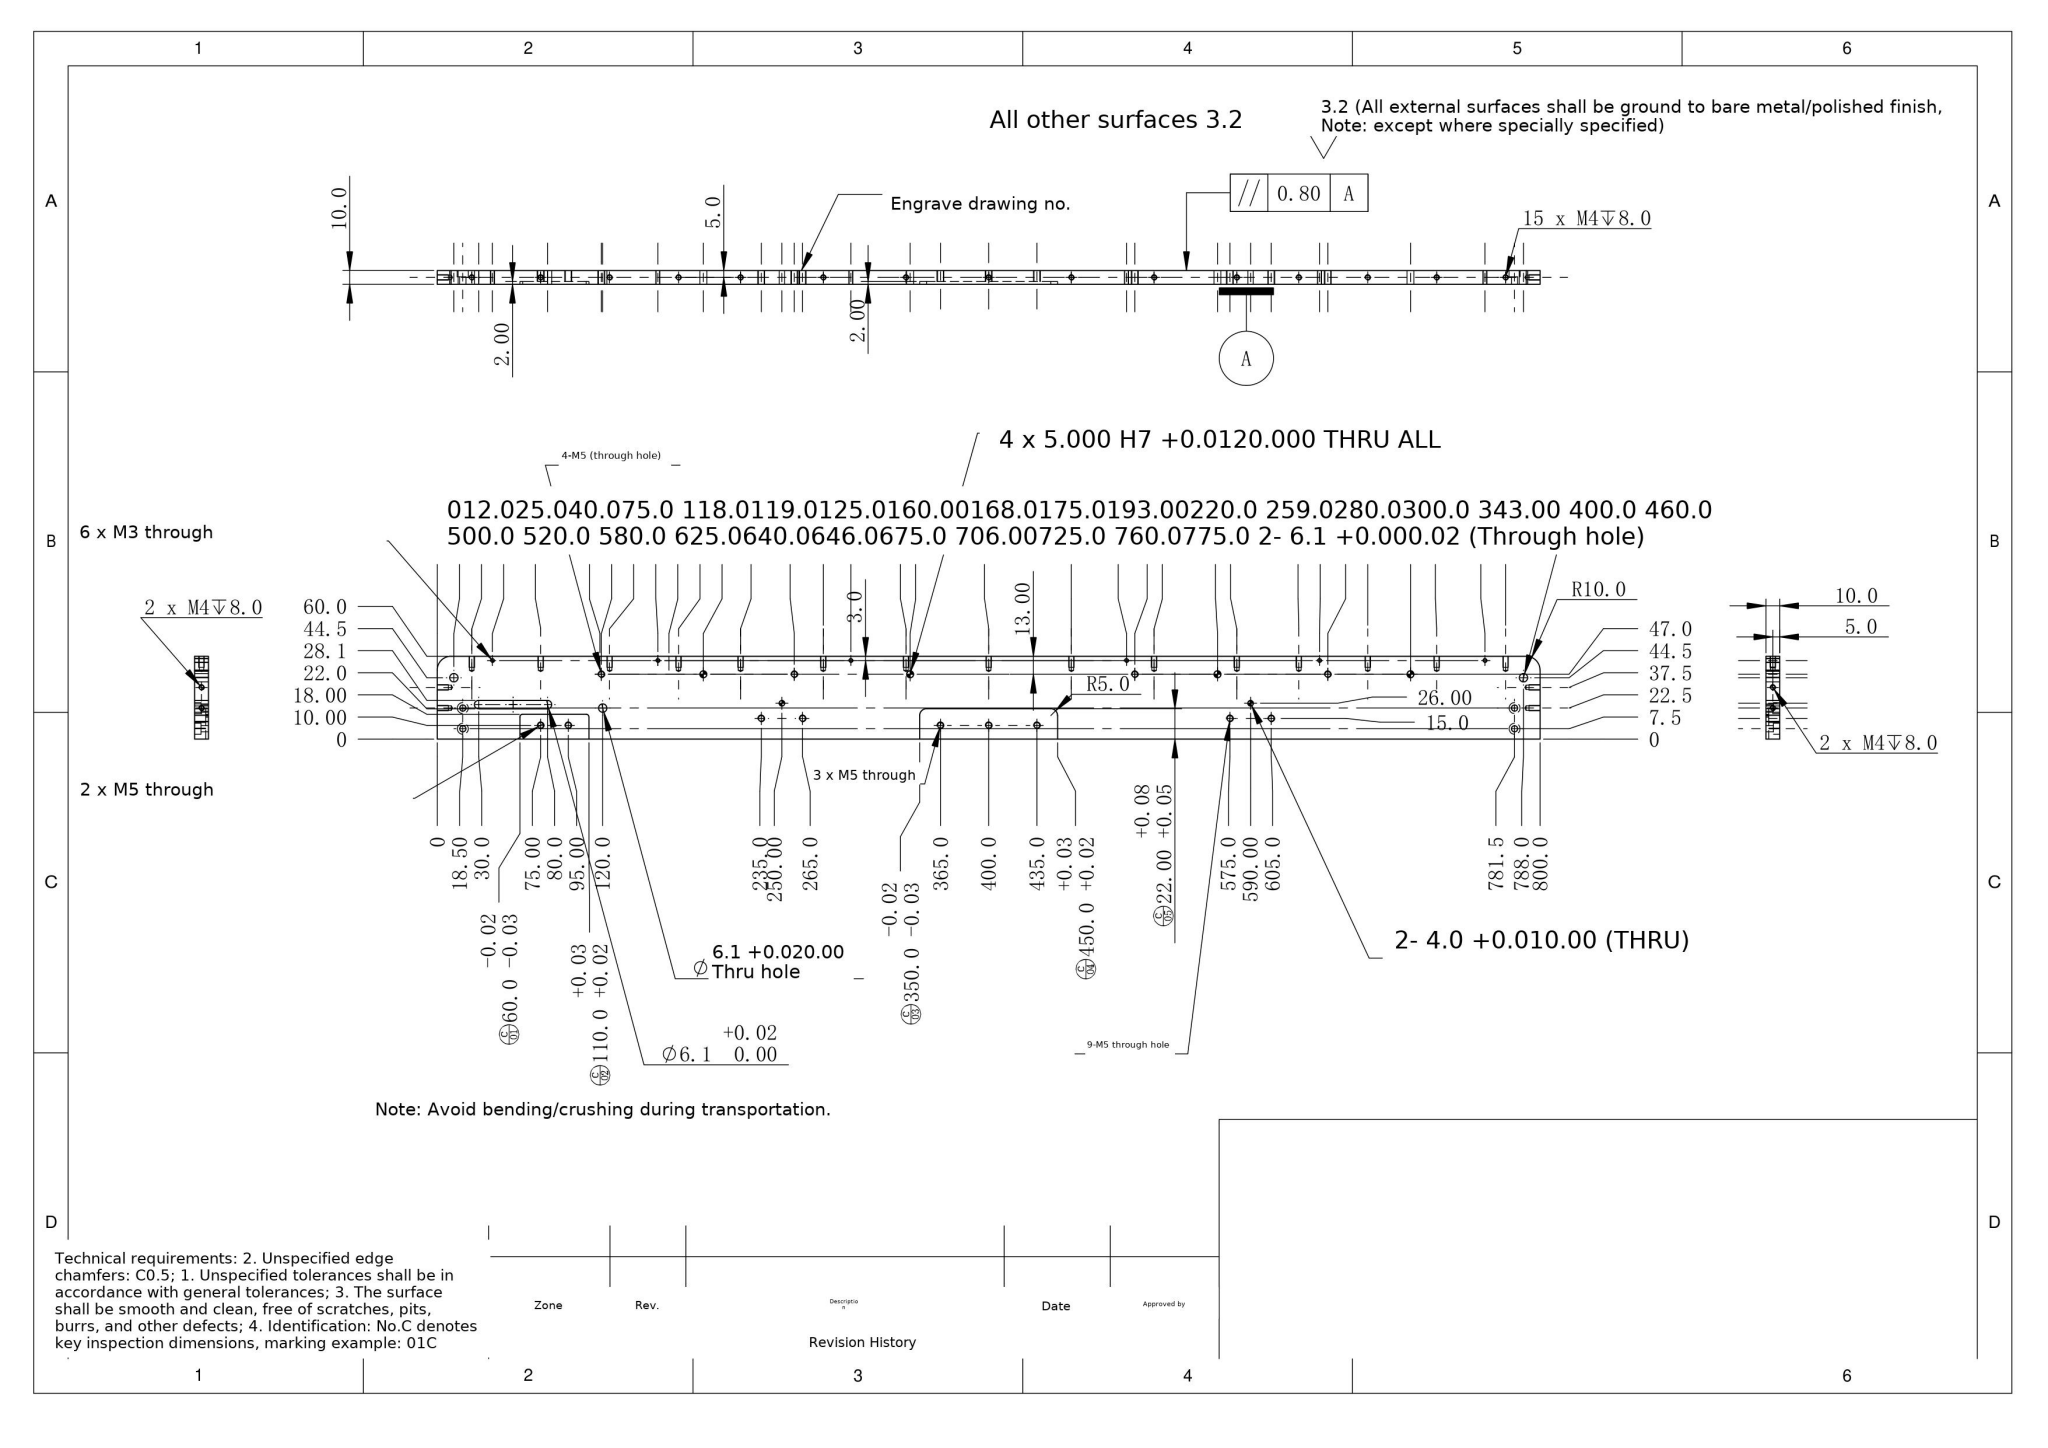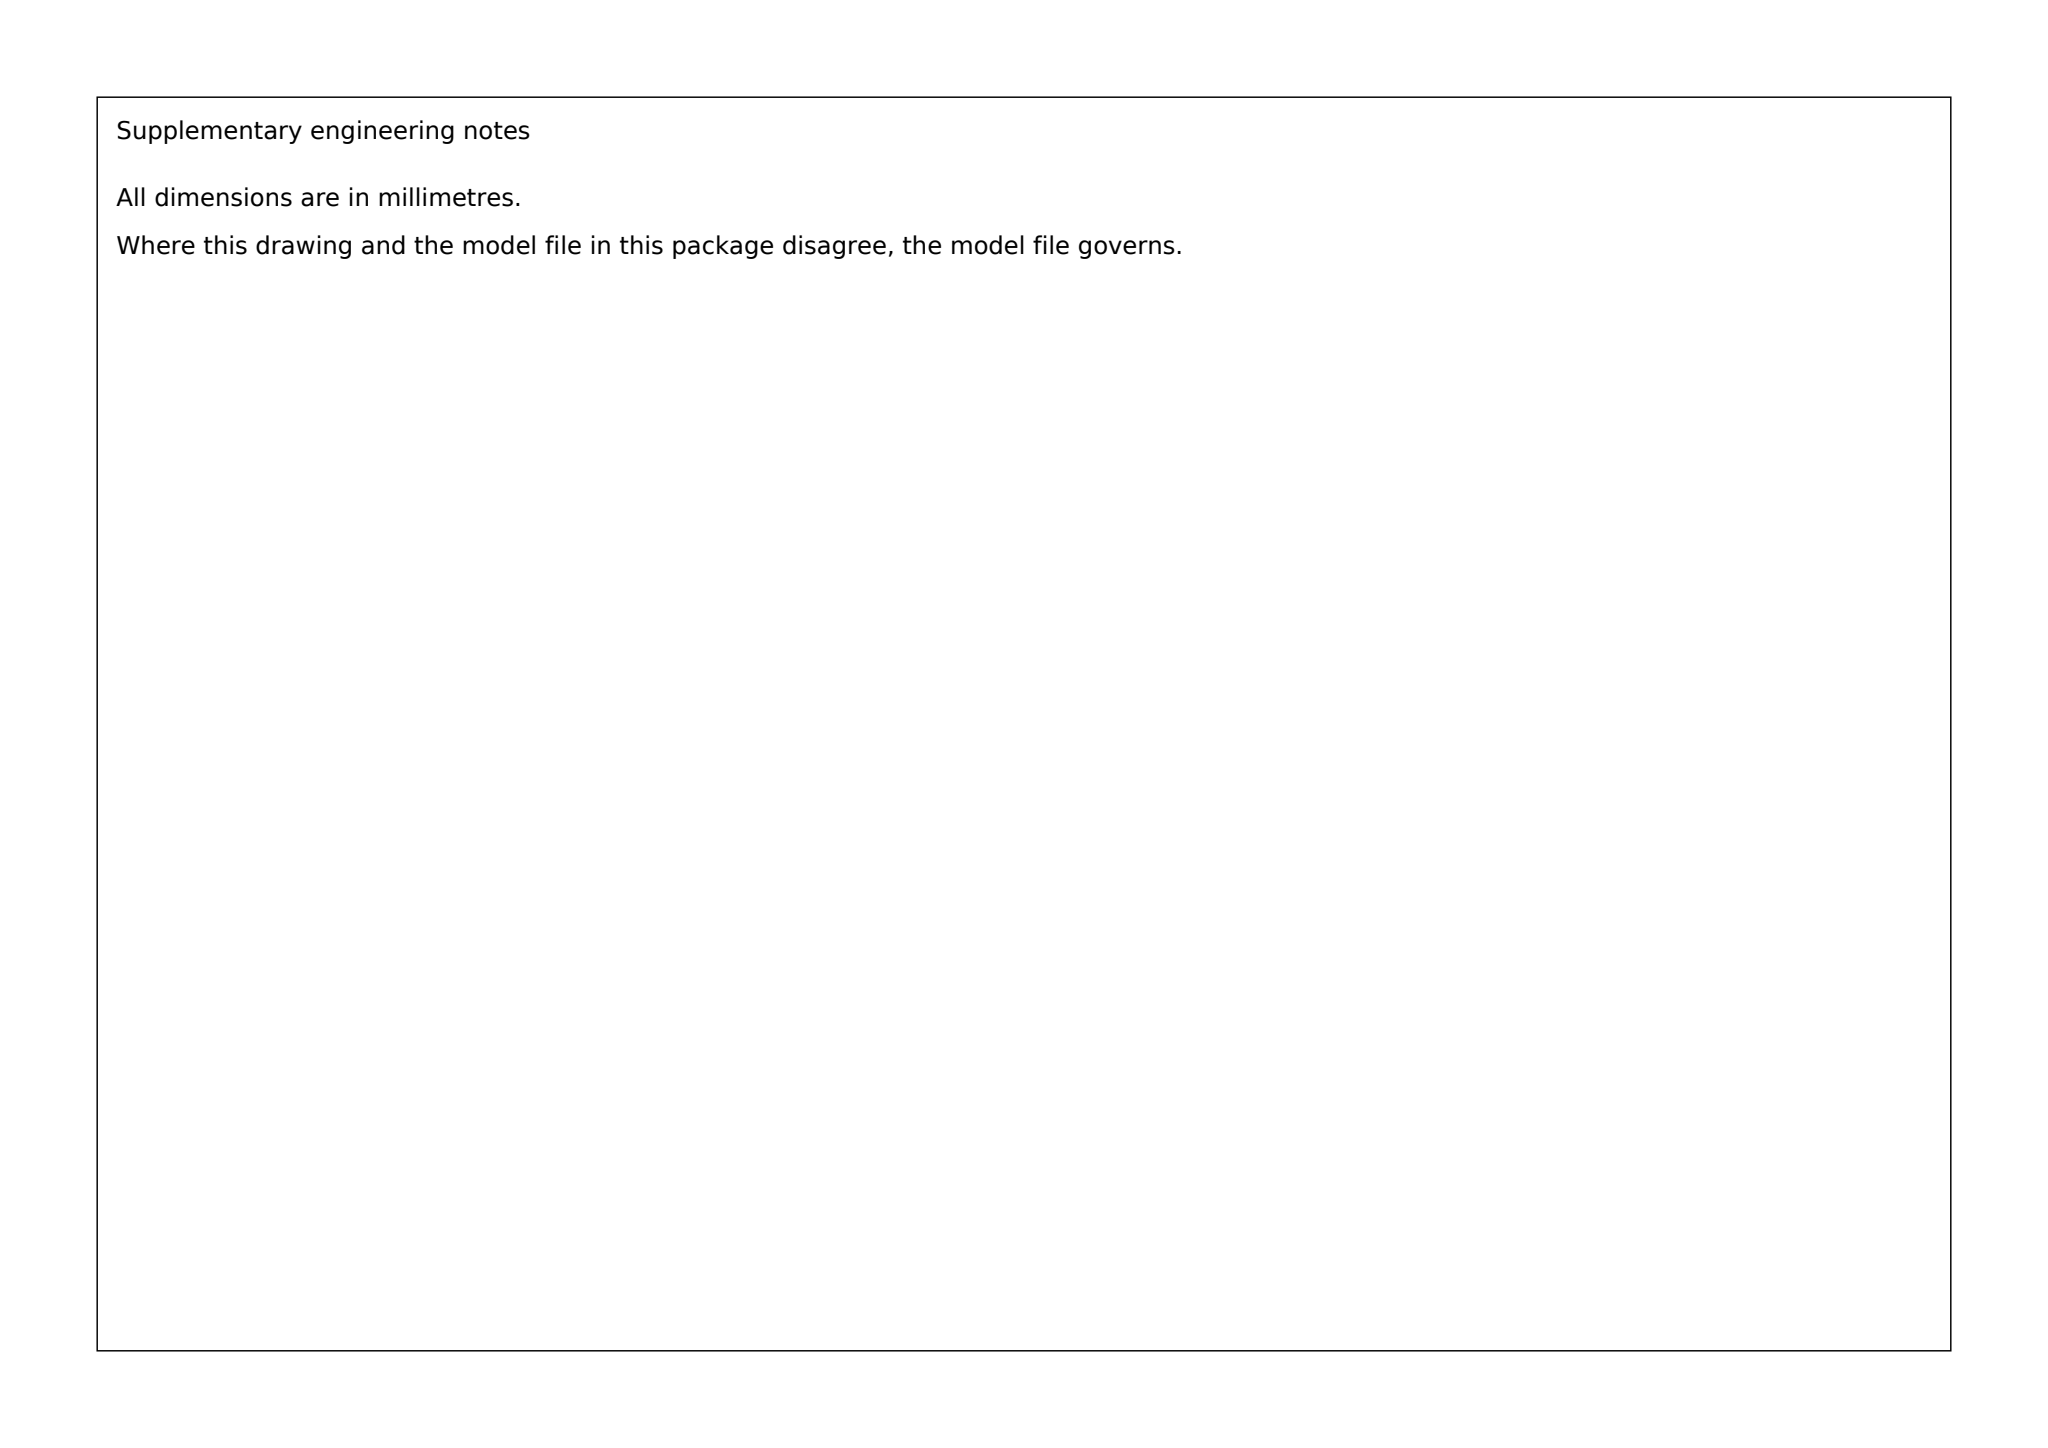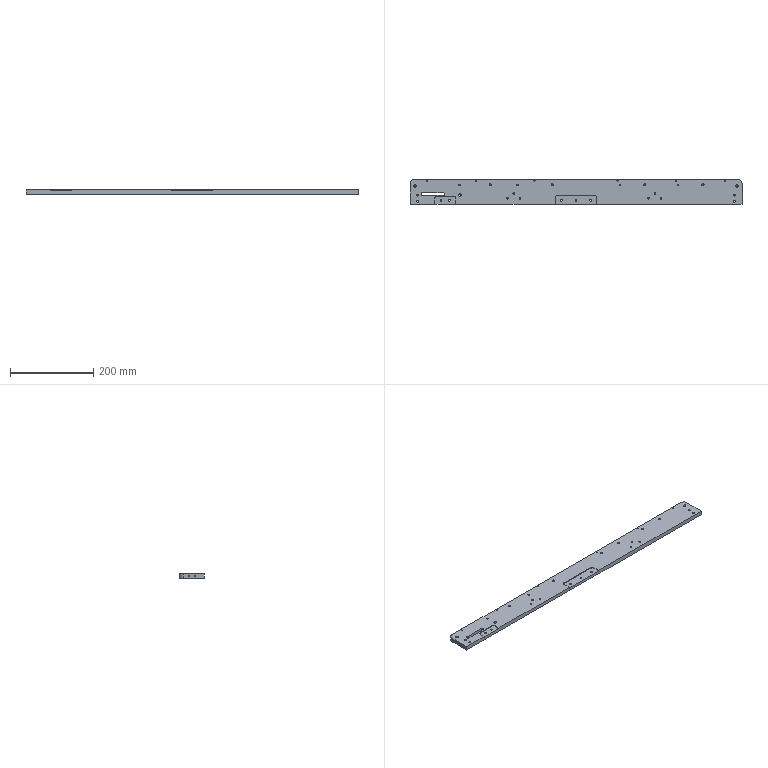Part | SolidWorks | mm | 1 solid | 177 faces | box 800 x 60 x 10 mm | volume 463219 mm3 | cylinder 119 | cone 38 | plane 20 | commonest cylinder face diameters 3.3 x38 4.2 x26 2.5 x12 6.1 x9 8 x8 4.5 x8 5 x8 4 x6
build123d program:
from build123d import *

# Parameters (mm, degrees)
SKETCH1_W                                         = 800
SKETCH1_H                                         = 60
BOSS_EXTRUDE1_DEPTH                               = 10
SKETCH2_R                                         = 3.05
CUT_EXTRUDE1_DEPTH                                = 803.309
SKETCH3_R                                         = 3.05
CUT_EXTRUDE2_DEPTH                                = 803.309
M5_TAPPED_HOLE1_D                                 = 4.2
LPATTERN1_COUNT                                   = 2
LPATTERN1_PITCH                                   = 30
M5_TAPPED_HOLE2_D                                 = 4.2
LPATTERN2_COUNT                                   = 2
LPATTERN2_PITCH                                   = 30
SKETCH10_R                                        = 3.05
CUT_EXTRUDE5_DEPTH                                = 803.309
M5_TAPPED_HOLE3_D                                 = 4.2
LPATTERN3_COUNT                                   = 2
LPATTERN3_PITCH                                   = 140
M5_TAPPED_HOLE4_D                                 = 4.2
LPATTERN4_COUNT                                   = 2
LPATTERN4_PITCH                                   = 140
SKETCH15_W                                        = 100
SKETCH15_H                                        = 22
CUT_EXTRUDE6_DEPTH                                = 2
FILLET1_R                                         = 5
FILLET2_R                                         = 10
M4_TAPPED_HOLE1_D                                 = 3.3
M4_TAPPED_HOLE1_DEPTH                             = 10.1
M4_TAPPED_HOLE1_TIP                               = 0.9914
M4_TAPPED_HOLE2_D                                 = 3.3
M4_TAPPED_HOLE2_DEPTH                             = 10.1
M4_TAPPED_HOLE2_TIP                               = 0.9914
F_4_0_4_DIAMETER_HOLE1_D                          = 4
M3_TAPPED_HOLE1_D                                 = 2.5
F_5_0_5_DIAMETER_HOLE1_D                          = 5
HOLE_SIZE_ACCORDING_TO_HEXAGON_SOCKET_D           = 4.5
HOLE_SIZE_ACCORDING_TO_HEXAGON_SOCKET_CBORE_D     = 8
HOLE_SIZE_ACCORDING_TO_HEXAGON_SOCKET_CBORE_DEPTH = 4.6
SKETCH34_W                                        = 50
SKETCH34_H                                        = 18
CUT_EXTRUDE7_DEPTH                                = 2
M5_TAPPED_HOLE5_D                                 = 4.2
FILLET3_R                                         = 2
M5_TAPPED_HOLE6_D                                 = 4.2
M4_TAPPED_HOLE3_D                                 = 3.3
M4_TAPPED_HOLE3_DEPTH                             = 10.1
M4_TAPPED_HOLE3_TIP                               = 0.9914
HOLE_SIZE_ACCORDING_TO_HEXAGON_SO_2_D             = 4.5
HOLE_SIZE_ACCORDING_TO_HEXAGON_SO_2_DEPTH         = 10.1
HOLE_SIZE_ACCORDING_TO_HEXAGON_SO_2_CBORE_D       = 8
HOLE_SIZE_ACCORDING_TO_HEXAGON_SO_2_CBORE_DEPTH   = 4.6
HOLE_SIZE_ACCORDING_TO_HEXAGON_SO_2_TIP           = 1.352
M4_TAPPED_HOLE4_D                                 = 3.3
M4_TAPPED_HOLE4_DEPTH                             = 10.1
M4_TAPPED_HOLE4_TIP                               = 0.9914


with BuildPart() as part:
    # Sketch1 → Boss-Extrude1 (new body)
    with BuildSketch(Plane.XY):
        with Locations((400, 30)):
            Rectangle(SKETCH1_W, SKETCH1_H)
    extrude(amount=BOSS_EXTRUDE1_DEPTH)

    # Sketch2 → Cut-Extrude1 (cut, through all)
    with BuildSketch(Plane(origin=(0, 0, 0), x_dir=(-1, 0, 0), z_dir=(0, 0, -1))):
        with Locations((-788, 44.5)):
            Circle(SKETCH2_R)
    extrude(amount=-CUT_EXTRUDE1_DEPTH, mode=Mode.SUBTRACT)

    # Sketch3 → Cut-Extrude2 (cut, through all)
    with BuildSketch(Plane(origin=(0, 0, 0), x_dir=(-1, 0, 0), z_dir=(0, 0, -1))):
        with Locations((-12, 44.5)):
            Circle(SKETCH3_R)
    extrude(amount=-CUT_EXTRUDE2_DEPTH, mode=Mode.SUBTRACT)

    # M5 Tapped Hole1 (through all)
    with Locations(Plane.XY.offset(10)):
        with Locations((235, 15)):
            m5_tapped_hole1 = Hole(M5_TAPPED_HOLE1_D / 2)

    # LPattern1: M5 Tapped Hole1 ×2
    with Locations(*[(i * LPATTERN1_PITCH, 0, 0) for i in range(1, LPATTERN1_COUNT)]):
        add(m5_tapped_hole1, mode=Mode.SUBTRACT)

    # M5 Tapped Hole2 (through all)
    with Locations(Plane.XY.offset(10)):
        with Locations((605, 15)):
            m5_tapped_hole2 = Hole(M5_TAPPED_HOLE2_D / 2)

    # LPattern2: M5 Tapped Hole2 ×2
    with Locations(*[(-i * LPATTERN2_PITCH, 0, 0) for i in range(1, LPATTERN2_COUNT)]):
        add(m5_tapped_hole2, mode=Mode.SUBTRACT)

    # Sketch10 → Cut-Extrude5 (cut, through all)
    with BuildSketch(Plane(origin=(0, 0, 0), x_dir=(-1, 0, 0), z_dir=(0, 0, -1))):
        with Locations((-120, 22.5)):
            Circle(SKETCH10_R)
        with BuildLine():
            Line((-80, 28.05), (-30, 28.05))
            ThreePointArc((-30, 28.05), (-26.95, 25), (-30, 21.95))
            Line((-30, 21.95), (-80, 21.95))
            ThreePointArc((-80, 21.95), (-83.05, 25), (-80, 28.05))
        make_face()
    extrude(amount=-CUT_EXTRUDE5_DEPTH, mode=Mode.SUBTRACT)

    # M5 Tapped Hole3 (through all)
    with Locations(Plane(origin=(0, 0, 0), x_dir=(-1, 0, 0), z_dir=(0, 0, -1))):
        with Locations((-646, 47)):
            m5_tapped_hole3 = Hole(M5_TAPPED_HOLE3_D / 2)

    # LPattern3: M5 Tapped Hole3 ×2
    with Locations(*[(-i * LPATTERN3_PITCH, 0, 0) for i in range(1, LPATTERN3_COUNT)]):
        add(m5_tapped_hole3, mode=Mode.SUBTRACT)

    # M5 Tapped Hole4 (through all)
    with Locations(Plane(origin=(0, 0, 0), x_dir=(-1, 0, 0), z_dir=(0, 0, -1))):
        with Locations((-119, 47)):
            m5_tapped_hole4 = Hole(M5_TAPPED_HOLE4_D / 2)

    # LPattern4: M5 Tapped Hole4 ×2
    with Locations(*[(i * LPATTERN4_PITCH, 0, 0) for i in range(1, LPATTERN4_COUNT)]):
        add(m5_tapped_hole4, mode=Mode.SUBTRACT)

    # Sketch15 → Cut-Extrude6 (cut)
    with BuildSketch(Plane.XY.offset(10)):
        with Locations((400, 11)):
            Rectangle(SKETCH15_W, SKETCH15_H)
    extrude(amount=-CUT_EXTRUDE6_DEPTH, mode=Mode.SUBTRACT)

    # Fillet1
    fillet1_edges = [part.edges().sort_by_distance(p)[0] for p in [
        (450, 22, 9),
        (350, 22, 9),
    ]]
    fillet(fillet1_edges, radius=FILLET1_R)

    # Fillet2
    fillet2_edges = [part.edges().sort_by_distance(p)[0] for p in [
        (0, 60, 5),
        (800, 60, 5),
    ]]
    fillet(fillet2_edges, radius=FILLET2_R)

    # M4 Tapped Hole1
    with Locations(Plane(origin=(0, 60, 0), x_dir=(1, 0, 0), z_dir=(0, 1, 0))):
        with Locations((775, -5), (725, -5), (25, -5), (75, -5), (675, -5), (625, -5), (125, -5), (175, -5)):
            Hole(M4_TAPPED_HOLE1_D / 2, depth=M4_TAPPED_HOLE1_DEPTH)
            with Locations((0, 0, -(M4_TAPPED_HOLE1_DEPTH + M4_TAPPED_HOLE1_TIP / 2))):  # 118° drill point
                Cone(0, M4_TAPPED_HOLE1_D / 2, M4_TAPPED_HOLE1_TIP, mode=Mode.SUBTRACT)

    # M4 Tapped Hole2
    with Locations(Plane(origin=(0, 60, 0), x_dir=(1, 0, 0), z_dir=(0, 1, 0))):
        with Locations((580, -5), (520, -5), (460, -5), (400, -5), (340, -5), (280, -5), (220, -5)):
            Hole(M4_TAPPED_HOLE2_D / 2, depth=M4_TAPPED_HOLE2_DEPTH)
            with Locations((0, 0, -(M4_TAPPED_HOLE2_DEPTH + M4_TAPPED_HOLE2_TIP / 2))):  # 118° drill point
                Cone(0, M4_TAPPED_HOLE2_D / 2, M4_TAPPED_HOLE2_TIP, mode=Mode.SUBTRACT)

    # 4.0 _4_ Diameter Hole1 (through all)
    with Locations(Plane.XY.offset(10)):
        with Locations((250, 26), (590, 26)):
            Hole(F_4_0_4_DIAMETER_HOLE1_D / 2)

    # M3 Tapped Hole1 (through all)
    with Locations(Plane.XY.offset(10)):
        with Locations((40, 57), (160, 57), (640, 57), (760, 57), (300, 57), (500, 57)):
            Hole(M3_TAPPED_HOLE1_D / 2)

    # 5.0 _5_ Diameter Hole1 (through all)
    with Locations(Plane(origin=(0, 0, 0), x_dir=(-1, 0, 0), z_dir=(0, 0, -1))):
        with Locations((-706, 47), (-566, 47), (-343, 47), (-193, 47)):
            Hole(F_5_0_5_DIAMETER_HOLE1_D / 2)

    # Hole Size _ according to_ Hexagon Socket (through all)
    with Locations(Plane(origin=(0, 0, 0), x_dir=(-1, 0, 0), z_dir=(0, 0, -1))):
        with Locations((-781.5, 22.5), (-781.5, 7.5)):
            CounterBoreHole(HOLE_SIZE_ACCORDING_TO_HEXAGON_SOCKET_D / 2, HOLE_SIZE_ACCORDING_TO_HEXAGON_SOCKET_CBORE_D / 2, HOLE_SIZE_ACCORDING_TO_HEXAGON_SOCKET_CBORE_DEPTH)

    # Sketch34 → Cut-Extrude7 (cut)
    with BuildSketch(Plane.XY.offset(10)):
        with Locations((85, 9)):
            Rectangle(SKETCH34_W, SKETCH34_H)
    extrude(amount=-CUT_EXTRUDE7_DEPTH, mode=Mode.SUBTRACT)

    # M5 Tapped Hole5 (through all)
    with Locations(Plane.XY.offset(8)):
        with Locations((75, 10), (95, 10)):
            Hole(M5_TAPPED_HOLE5_D / 2)

    # Fillet3
    fillet3_edges = [part.edges().sort_by_distance(p)[0] for p in [
        (60, 18, 9),
        (110, 18, 9),
    ]]
    fillet(fillet3_edges, radius=FILLET3_R)

    # M5 Tapped Hole6 (through all)
    with Locations(Plane.XY.offset(8)):
        with Locations((365, 10), (400, 10), (435, 10)):
            Hole(M5_TAPPED_HOLE6_D / 2)

    # M4 Tapped Hole3
    with Locations(Plane(origin=(800, 0, 0), x_dir=(0, 0, -1), z_dir=(1, 0, 0))):
        with Locations((-5, 37.5), (-5, 22.5)):
            Hole(M4_TAPPED_HOLE3_D / 2, depth=M4_TAPPED_HOLE3_DEPTH)
            with Locations((0, 0, -(M4_TAPPED_HOLE3_DEPTH + M4_TAPPED_HOLE3_TIP / 2))):  # 118° drill point
                Cone(0, M4_TAPPED_HOLE3_D / 2, M4_TAPPED_HOLE3_TIP, mode=Mode.SUBTRACT)

    # Hole Size _ according to_ Hexagon So 2
    with Locations(Plane(origin=(0, 0, 0), x_dir=(-1, 0, 0), z_dir=(0, 0, -1))):
        with Locations((-18.5, 22.5), (-18.5, 7.5)):
            CounterBoreHole(HOLE_SIZE_ACCORDING_TO_HEXAGON_SO_2_D / 2, HOLE_SIZE_ACCORDING_TO_HEXAGON_SO_2_CBORE_D / 2, HOLE_SIZE_ACCORDING_TO_HEXAGON_SO_2_CBORE_DEPTH, depth=HOLE_SIZE_ACCORDING_TO_HEXAGON_SO_2_DEPTH)
            with Locations((0, 0, -(HOLE_SIZE_ACCORDING_TO_HEXAGON_SO_2_DEPTH + HOLE_SIZE_ACCORDING_TO_HEXAGON_SO_2_TIP / 2))):  # 118° drill point
                Cone(0, HOLE_SIZE_ACCORDING_TO_HEXAGON_SO_2_D / 2, HOLE_SIZE_ACCORDING_TO_HEXAGON_SO_2_TIP, mode=Mode.SUBTRACT)

    # M4 Tapped Hole4
    with Locations(Plane.ZY):
        with Locations((5, 37.5), (5, 22.5)):
            Hole(M4_TAPPED_HOLE4_D / 2, depth=M4_TAPPED_HOLE4_DEPTH)
            with Locations((0, 0, -(M4_TAPPED_HOLE4_DEPTH + M4_TAPPED_HOLE4_TIP / 2))):  # 118° drill point
                Cone(0, M4_TAPPED_HOLE4_D / 2, M4_TAPPED_HOLE4_TIP, mode=Mode.SUBTRACT)


solid = part.part